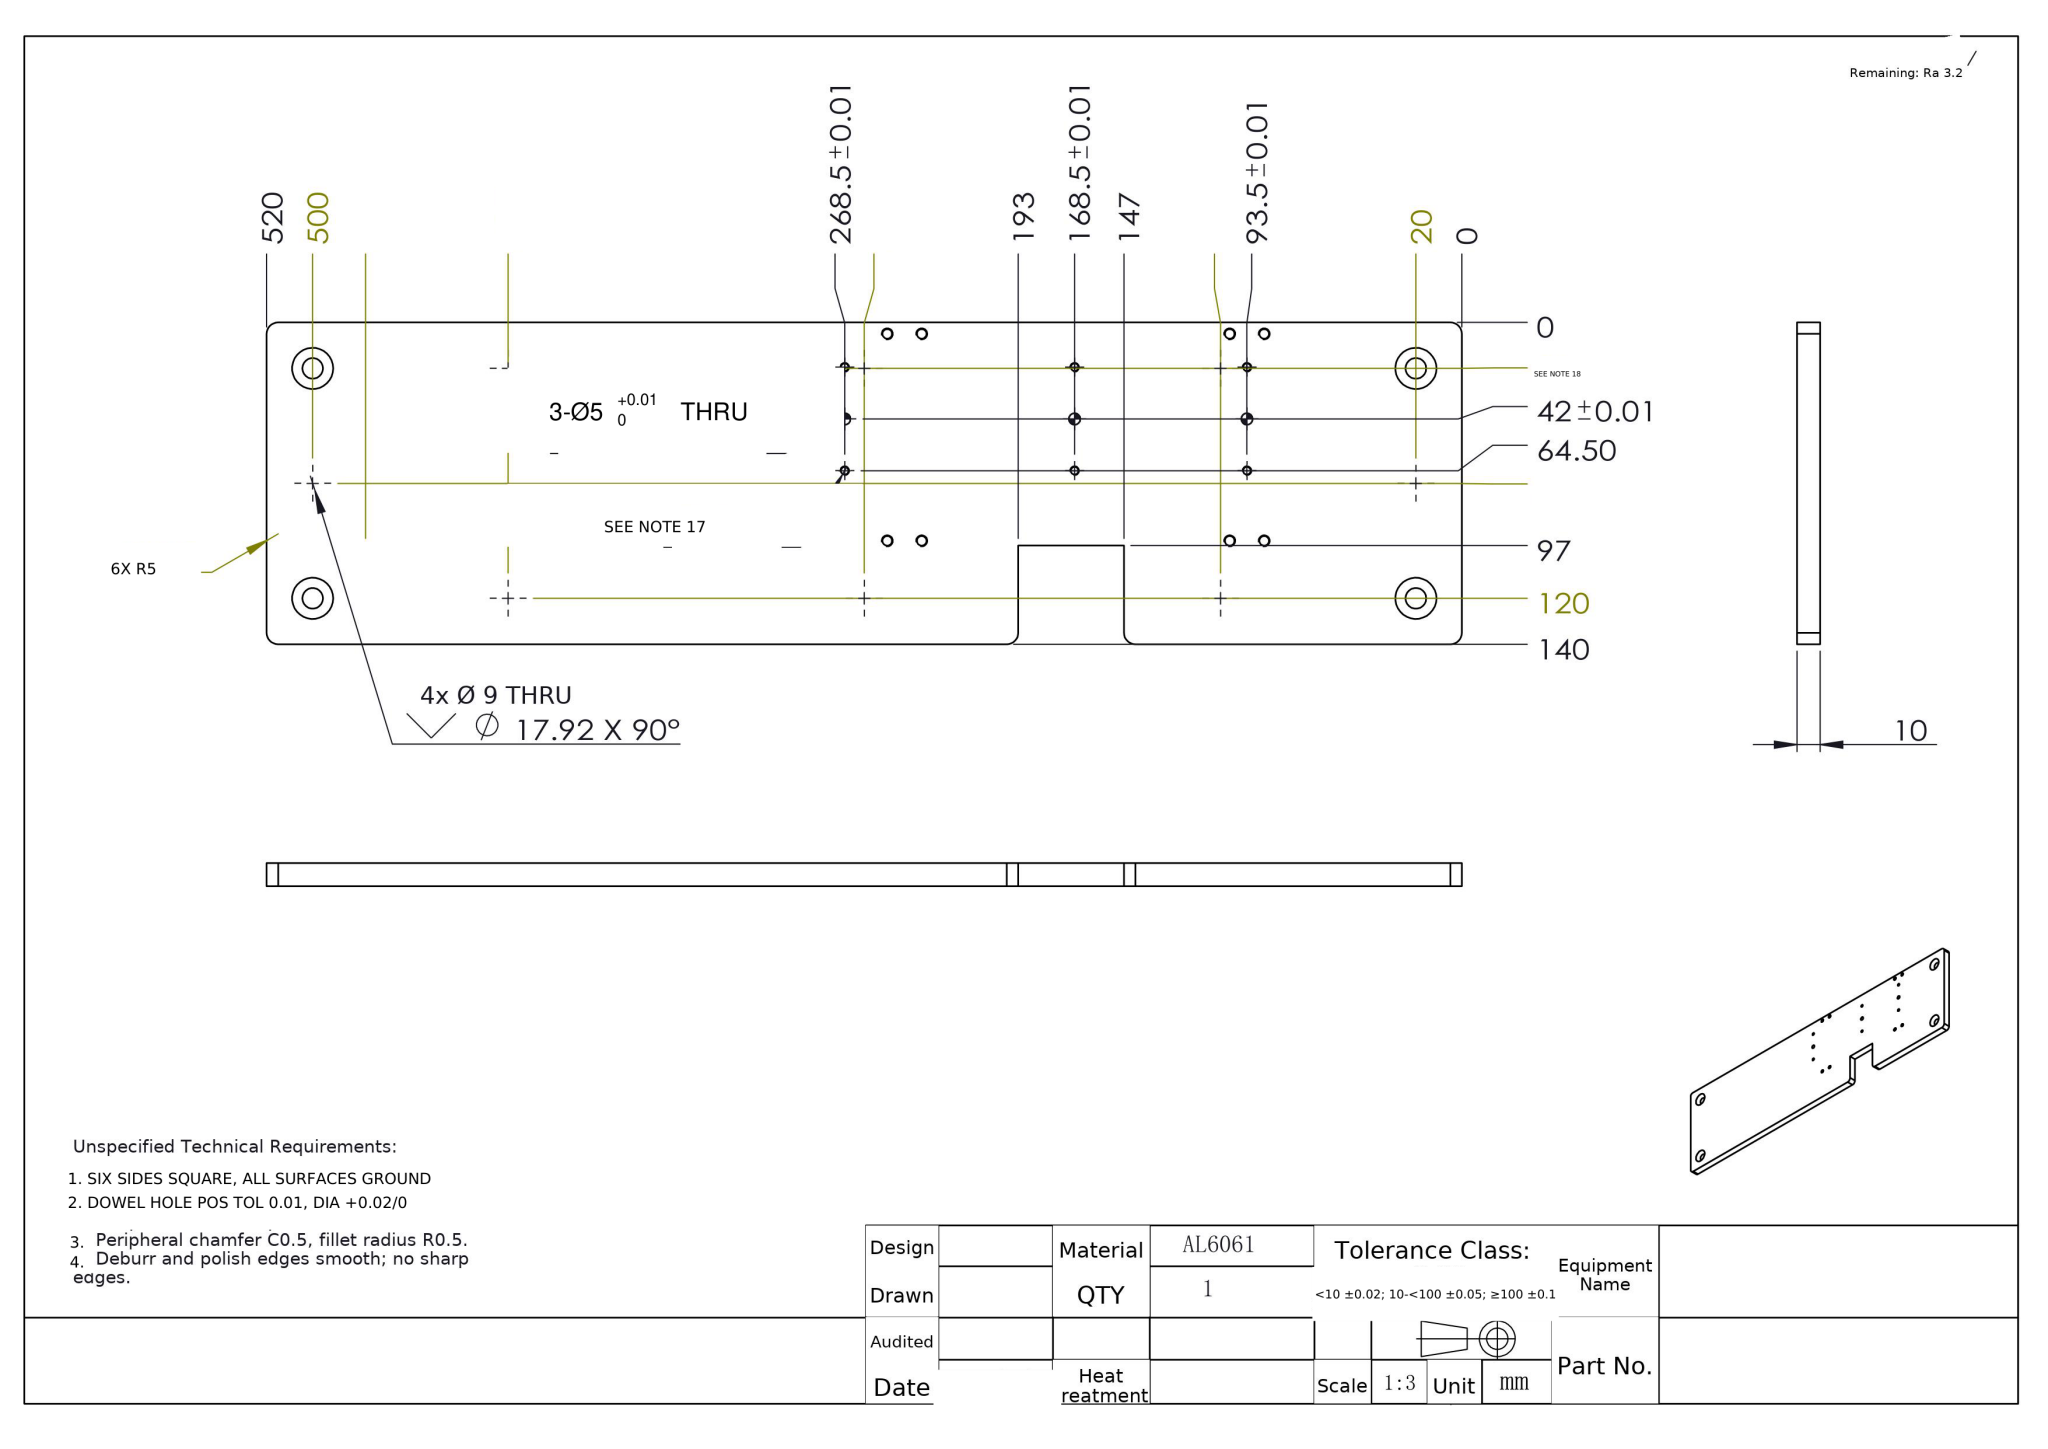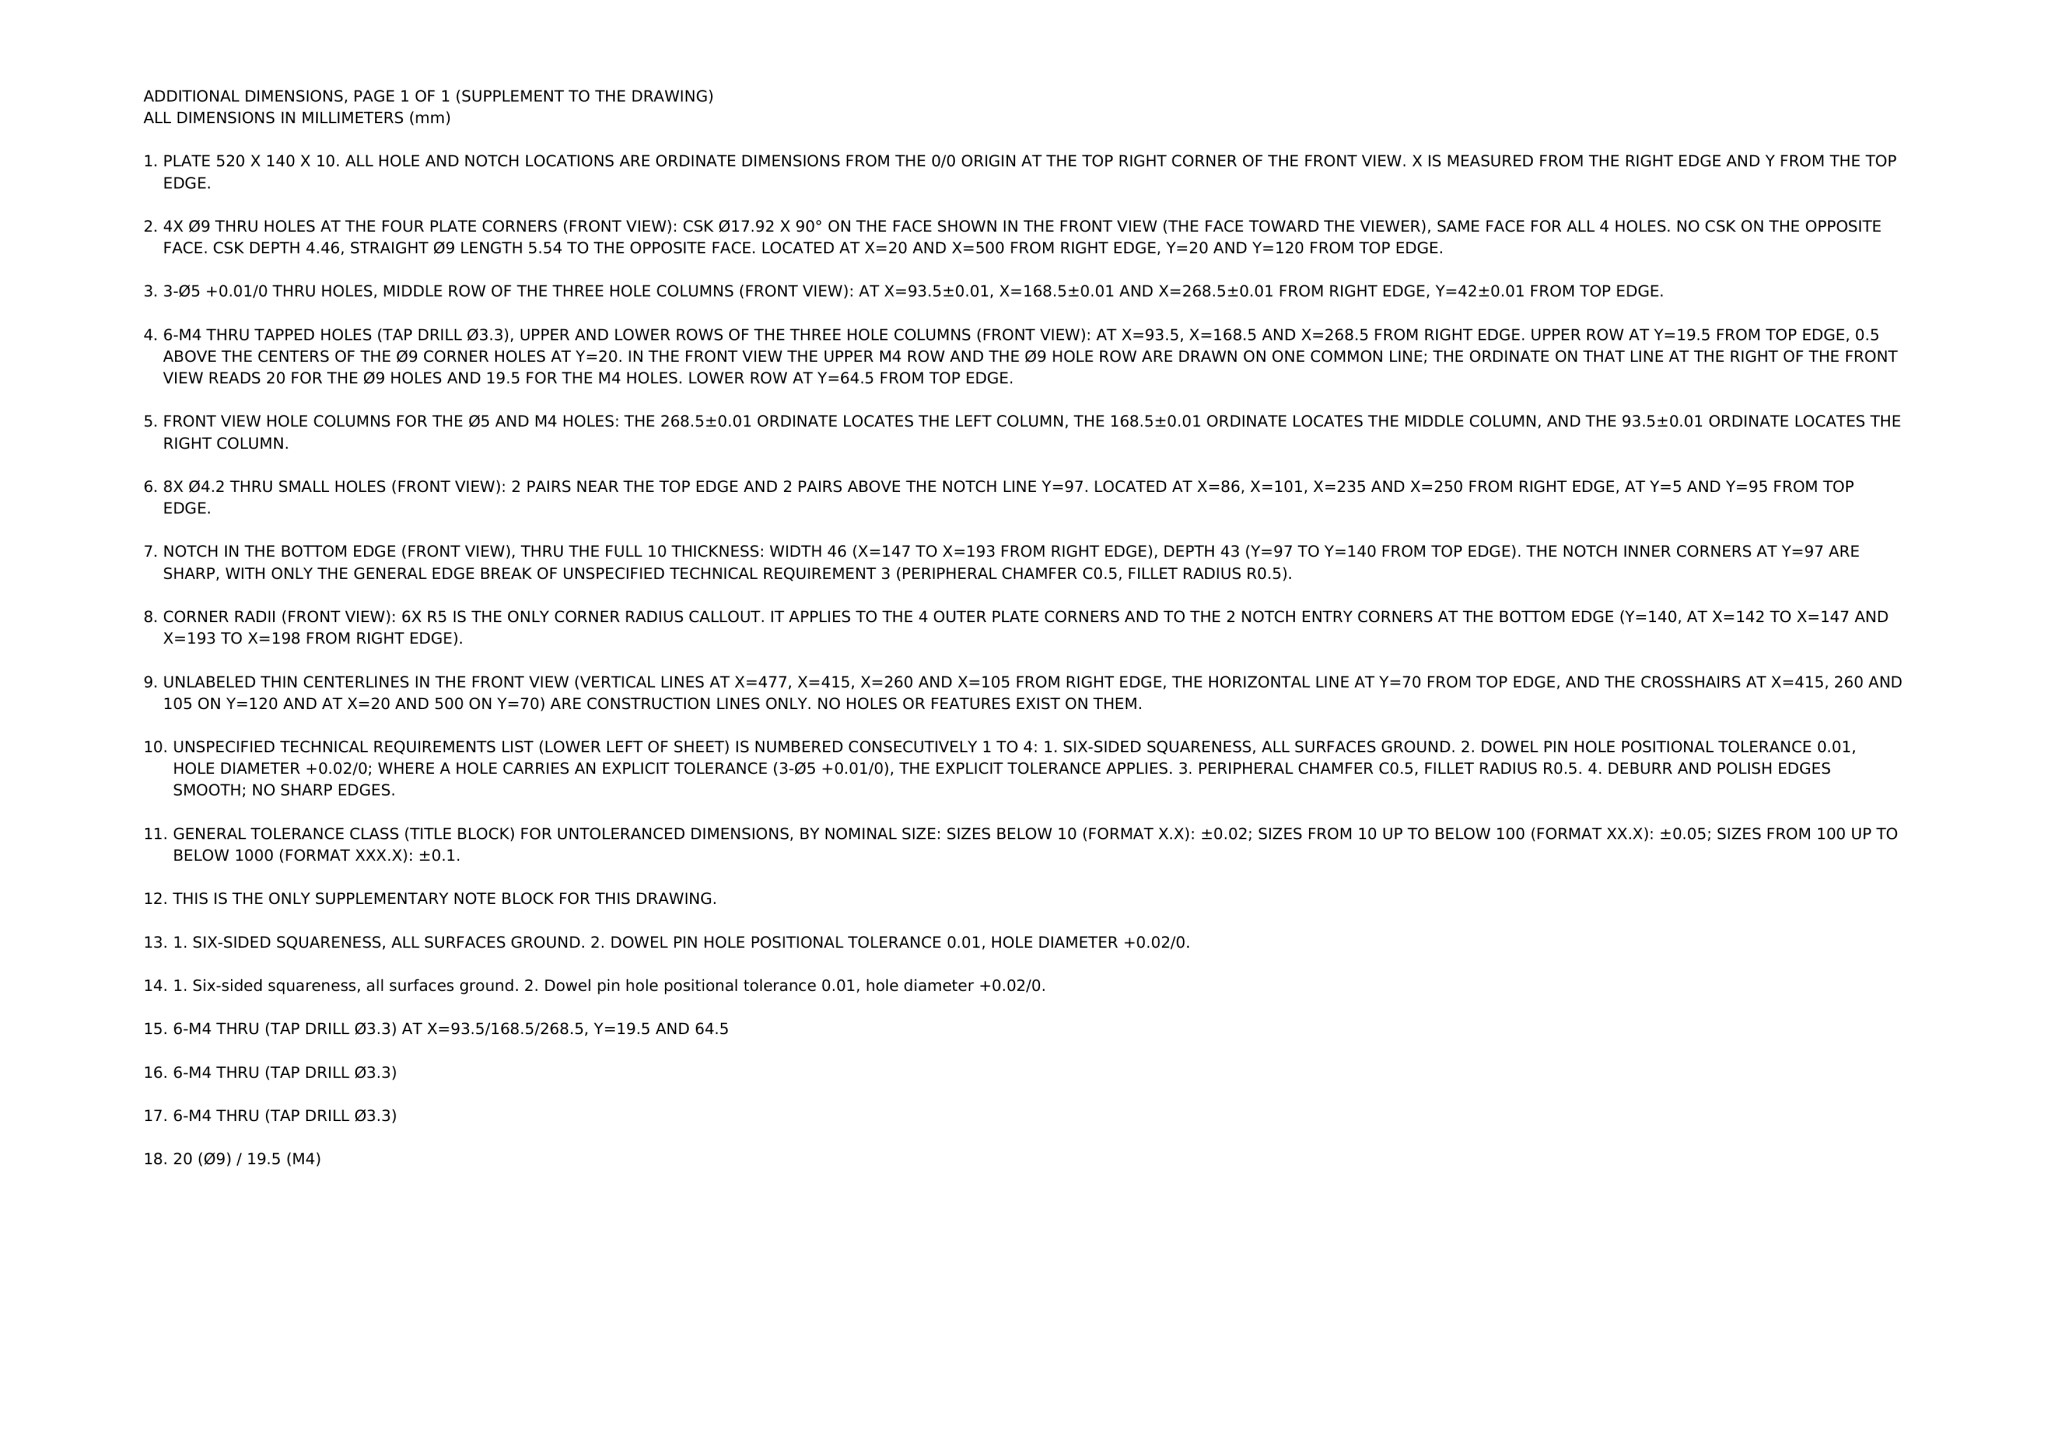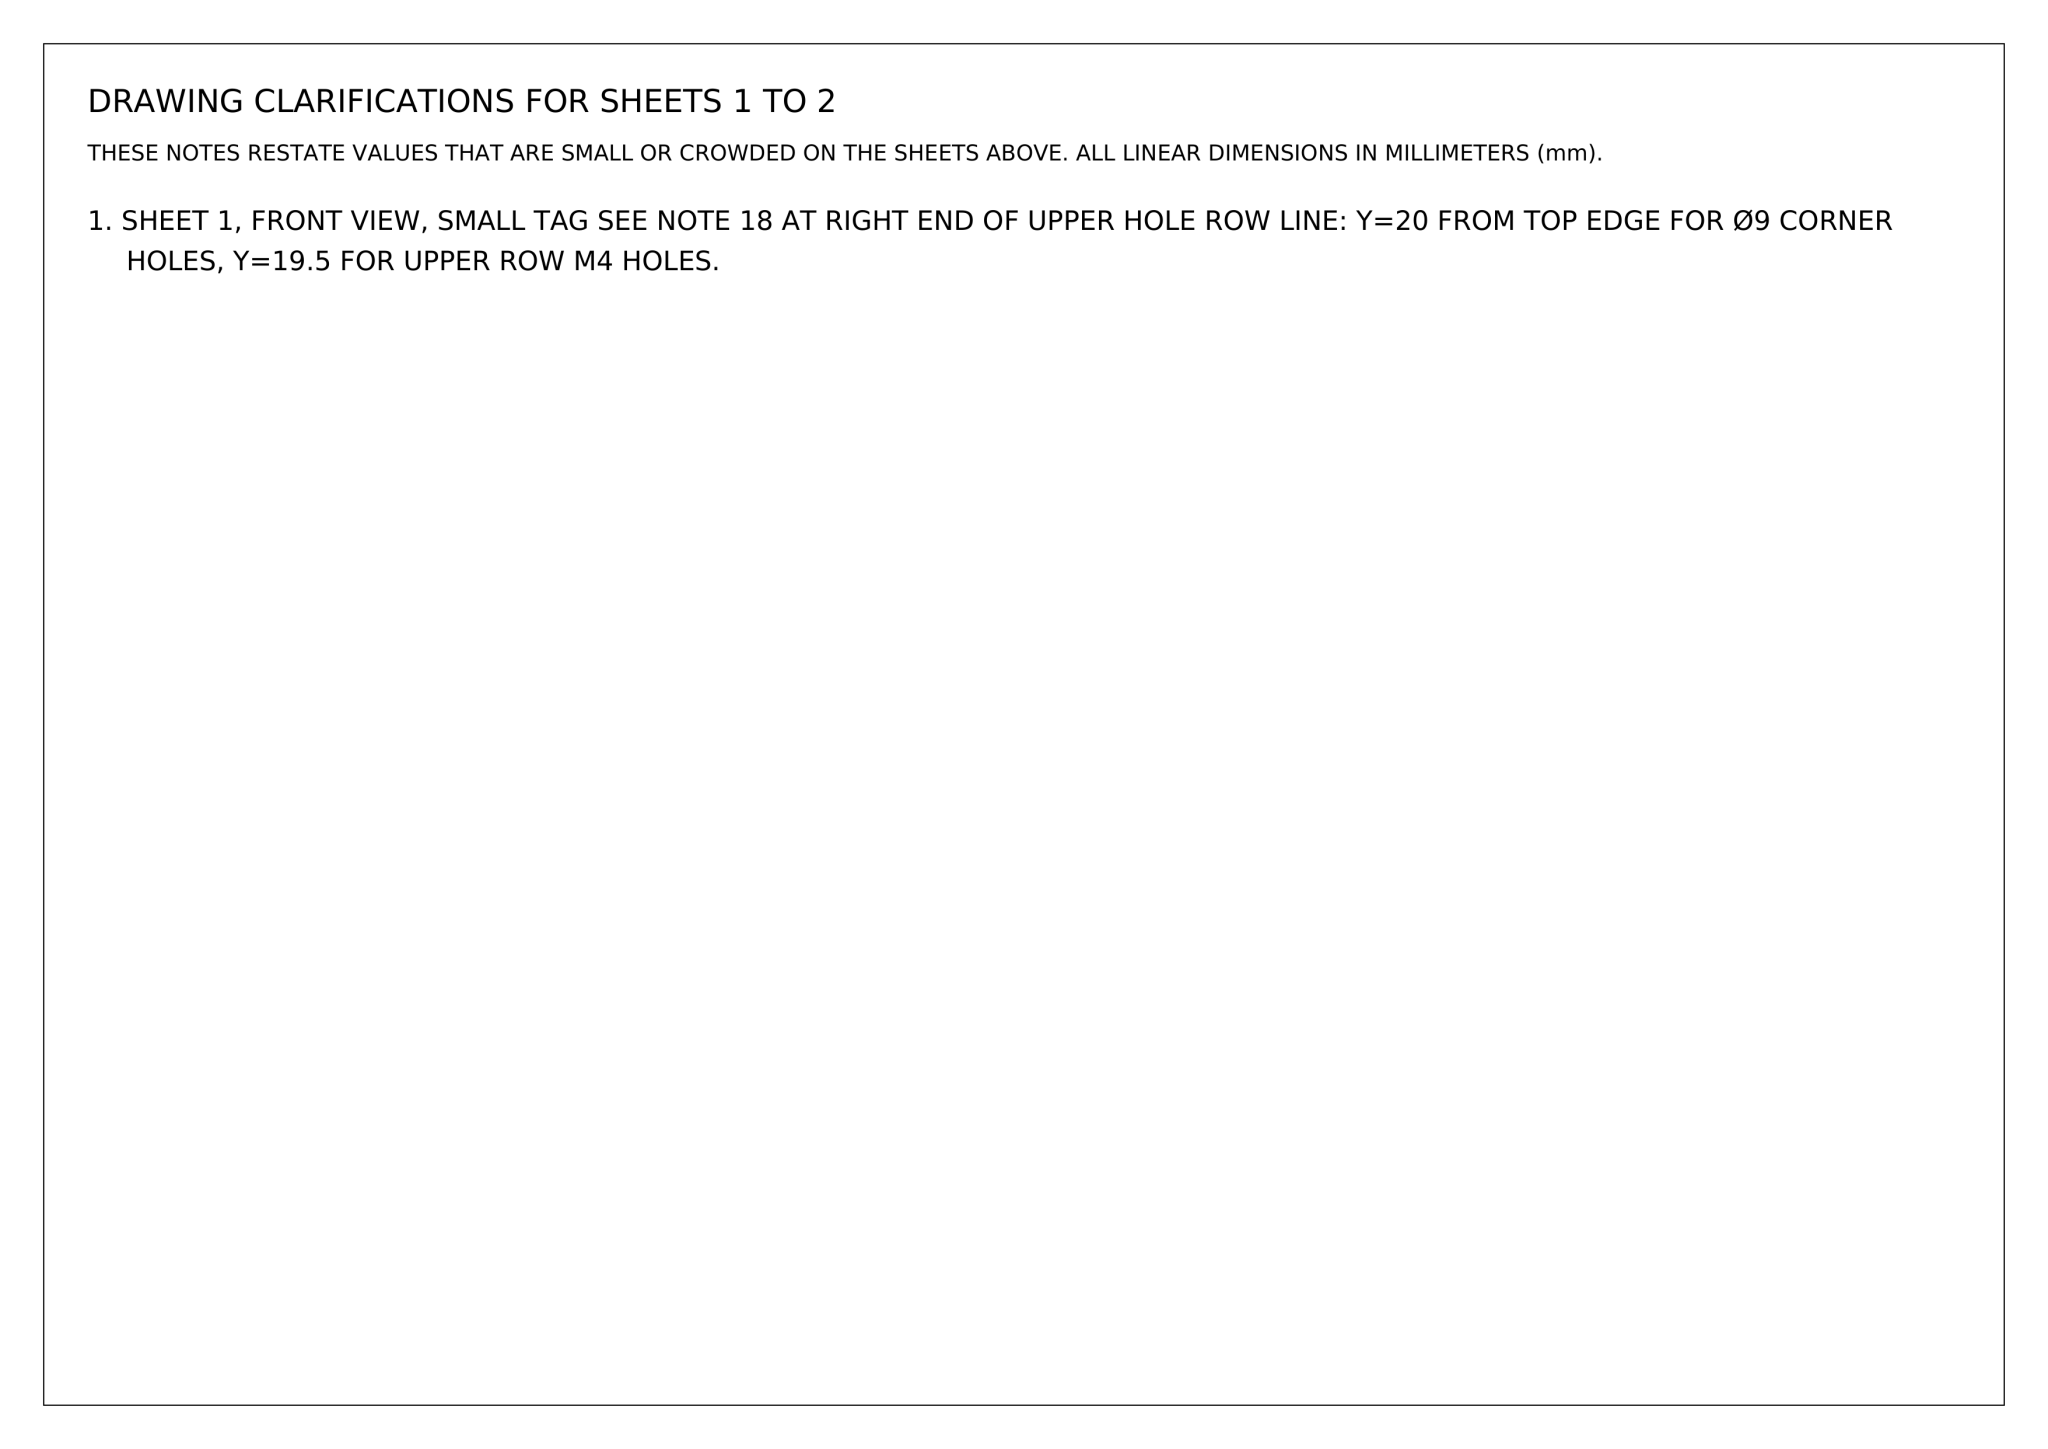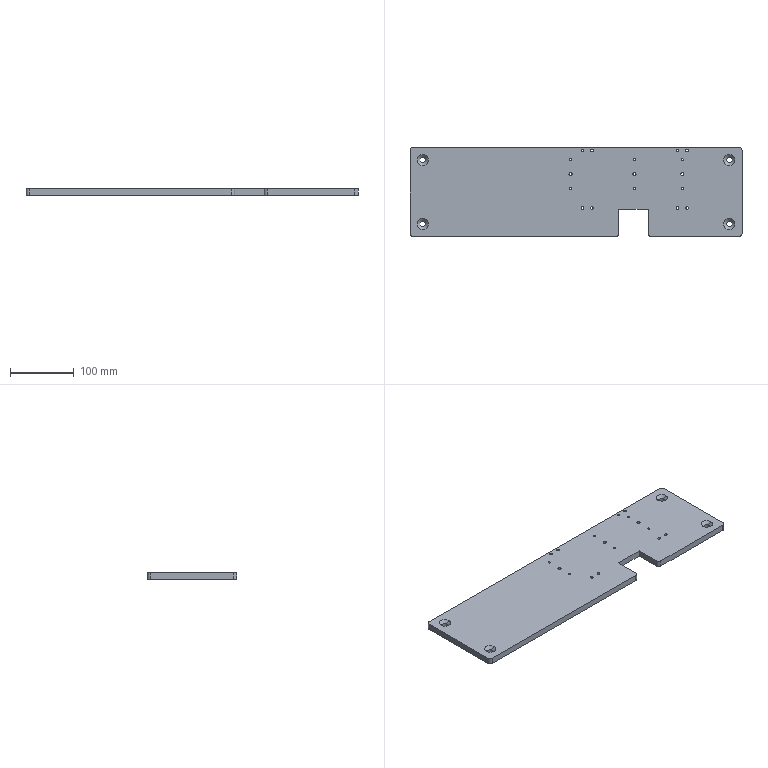Part | NX | mm | 1 solid | 66 faces | box 520 x 140 x 10 mm | volume 701646 mm3 | cylinder 48 | plane 10 | cone 8 | commonest cylinder face diameters 4.2 x16 3.3 x12 9 x8 5 x6 10 x6